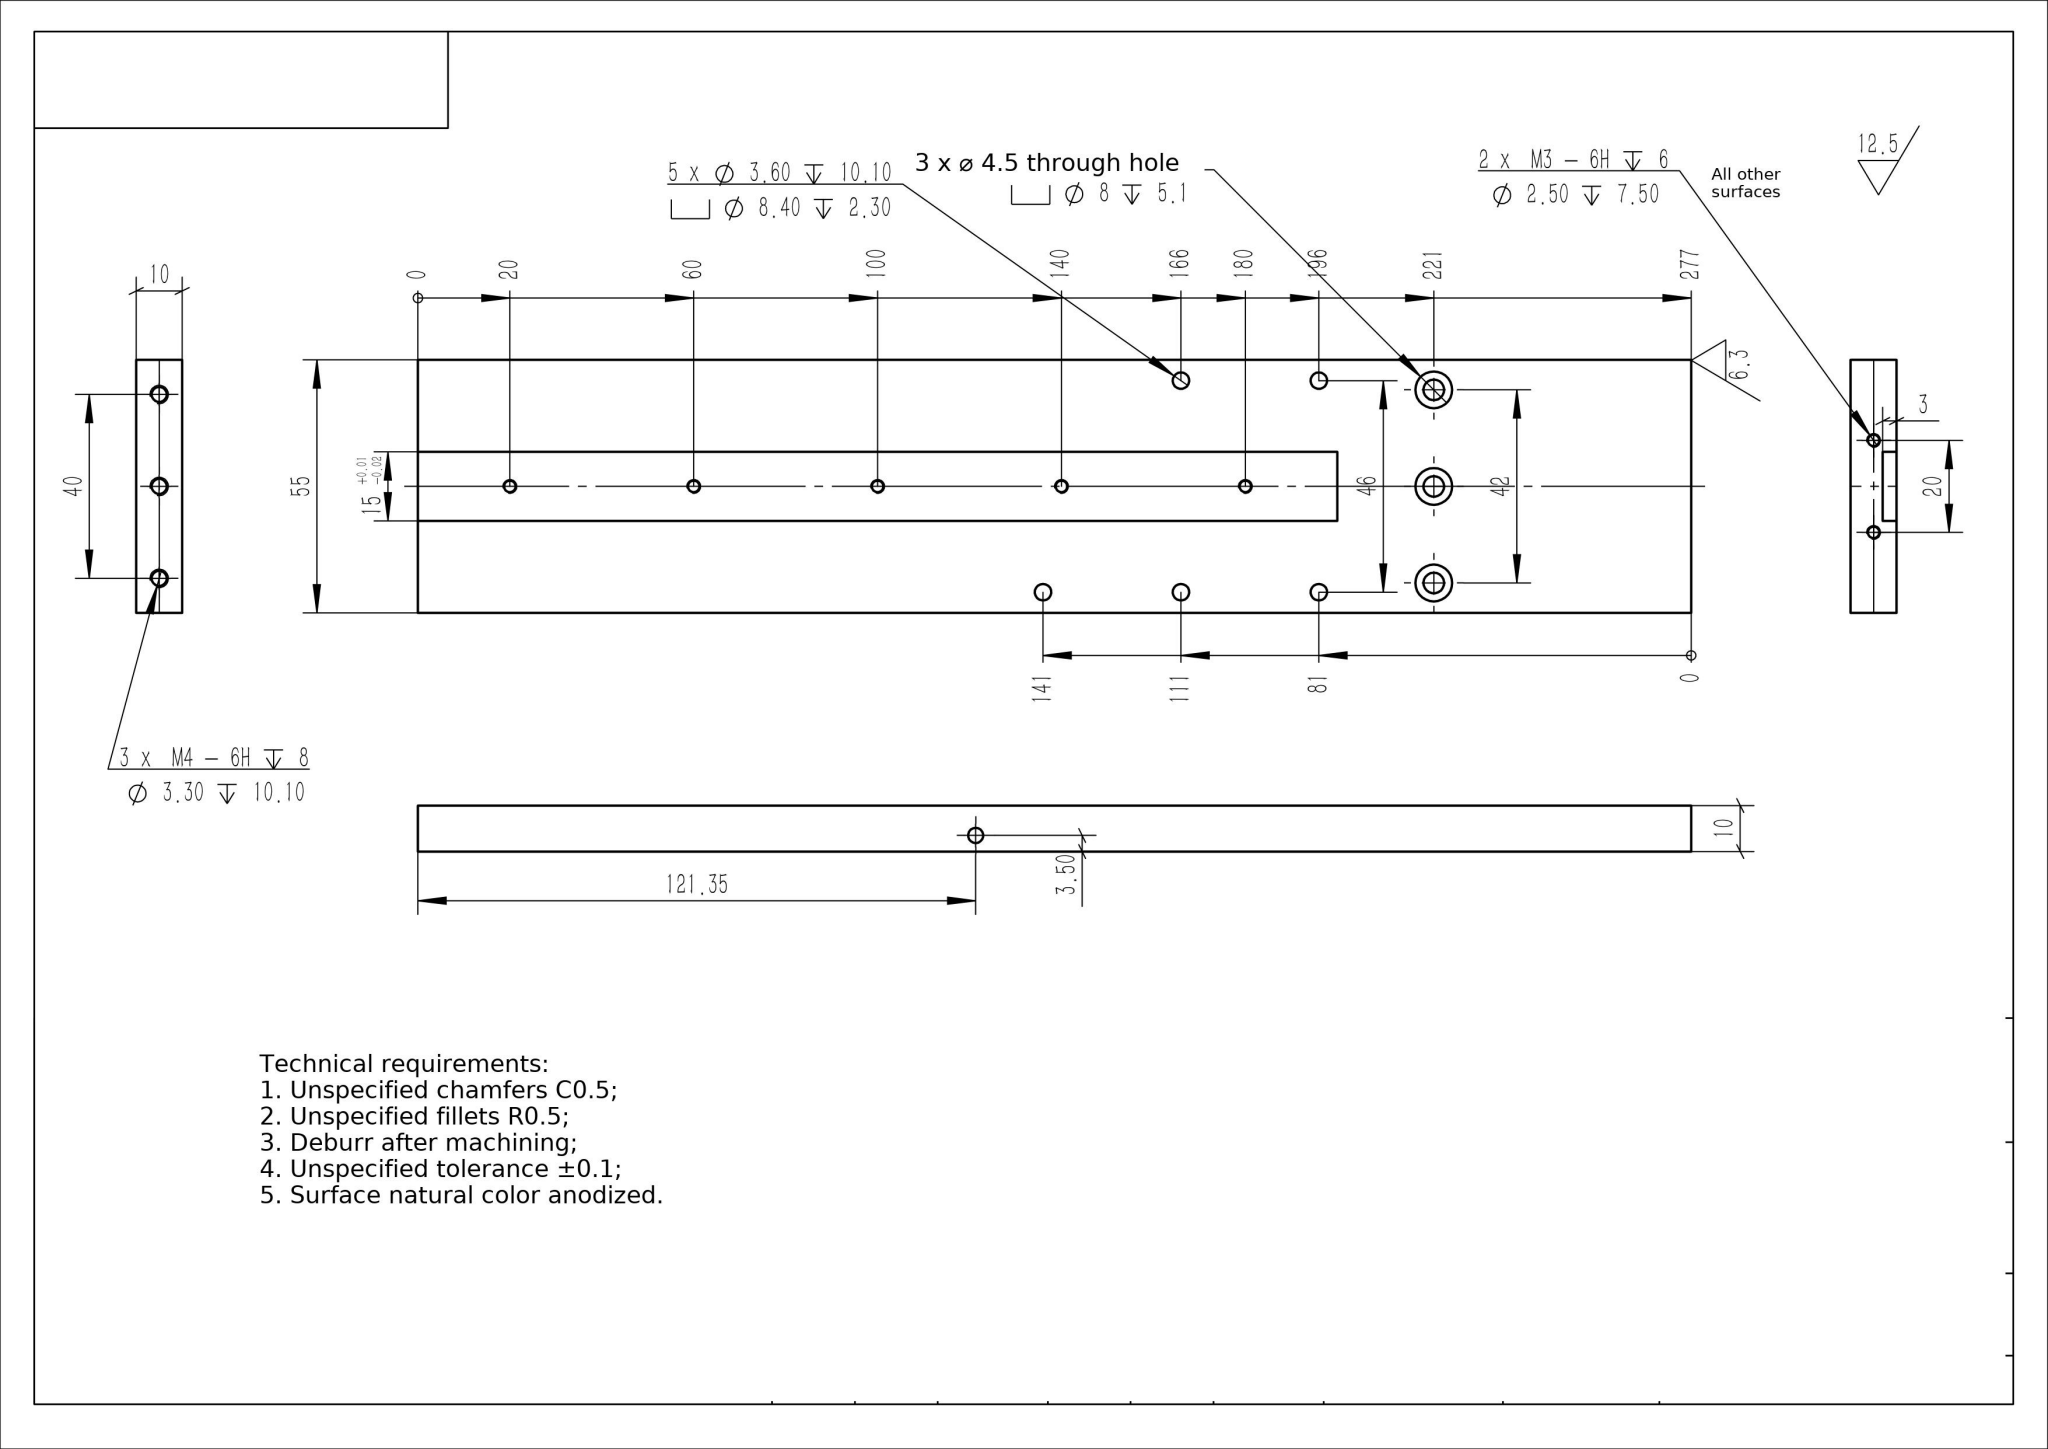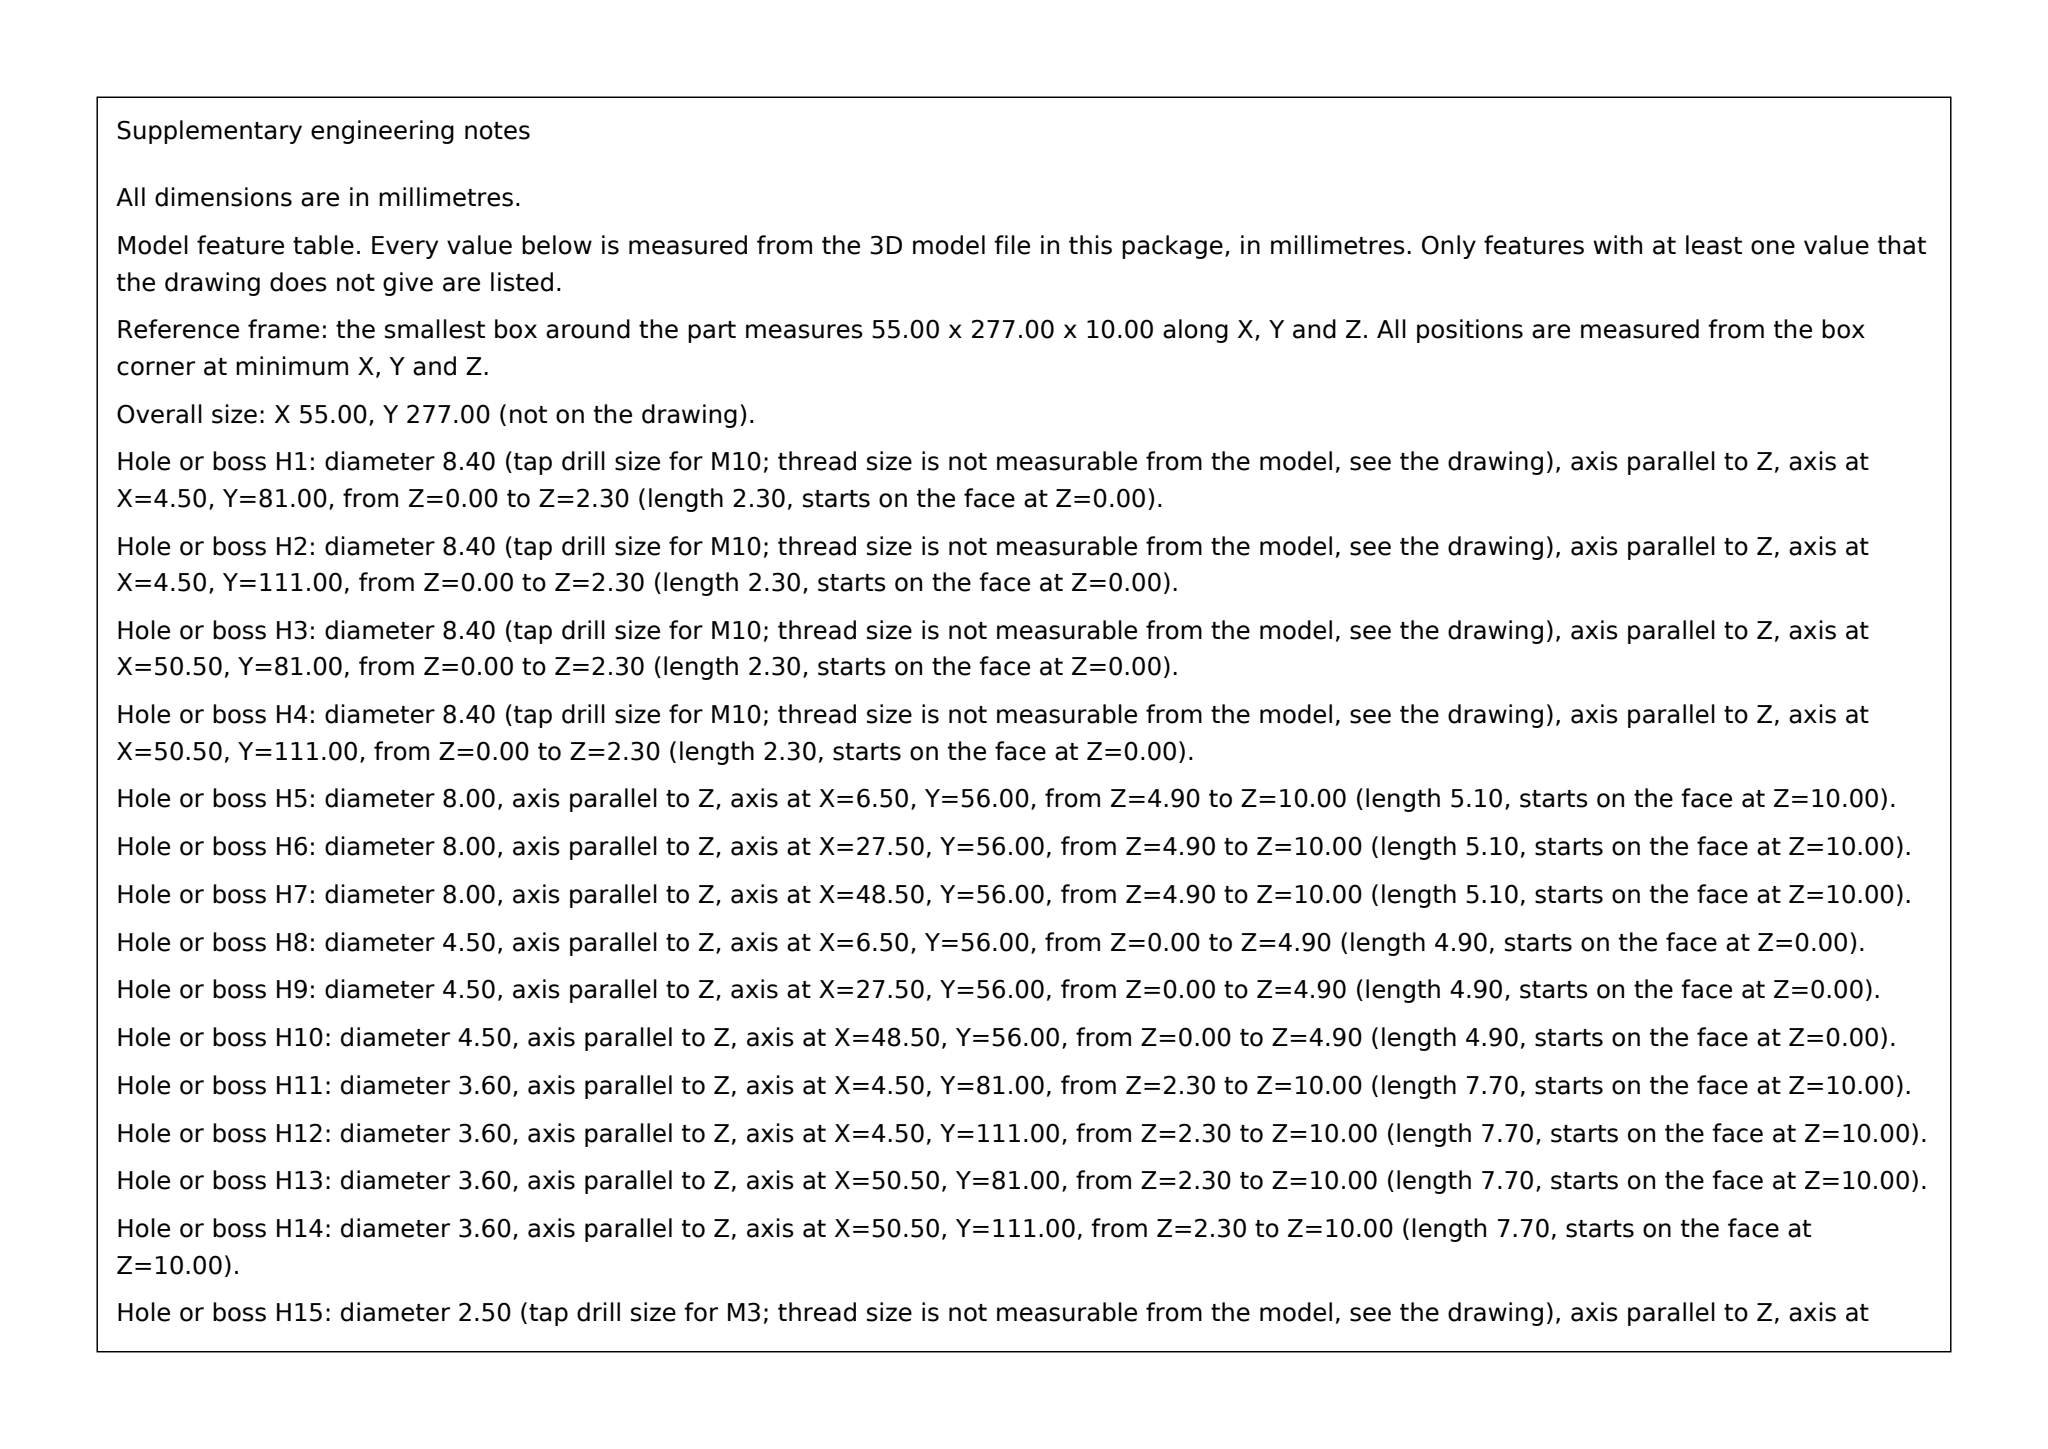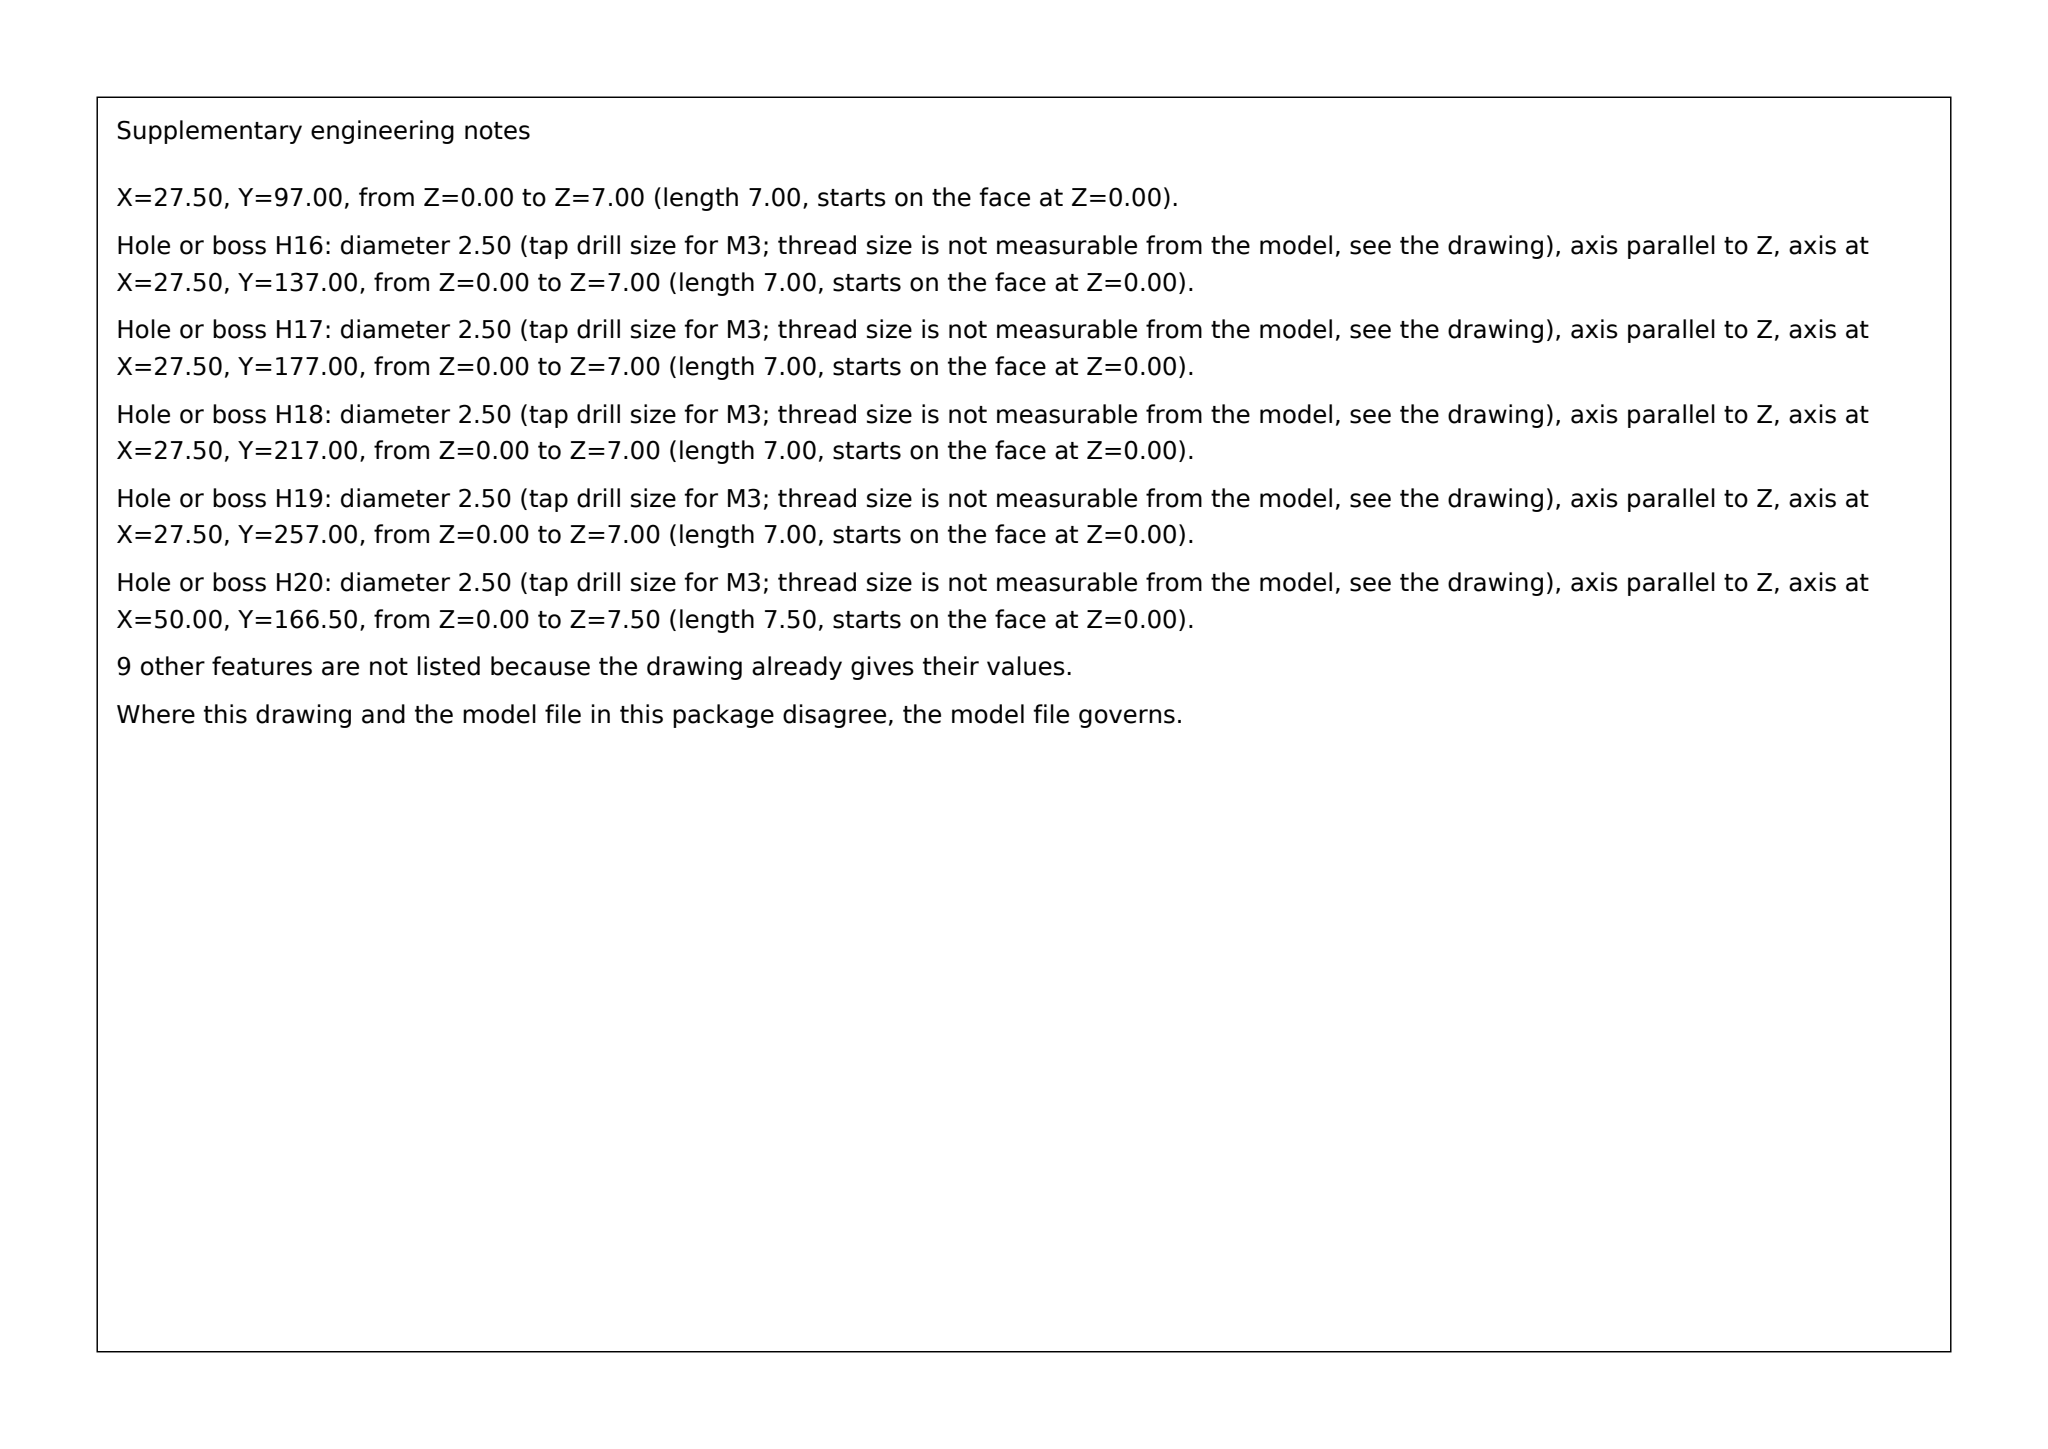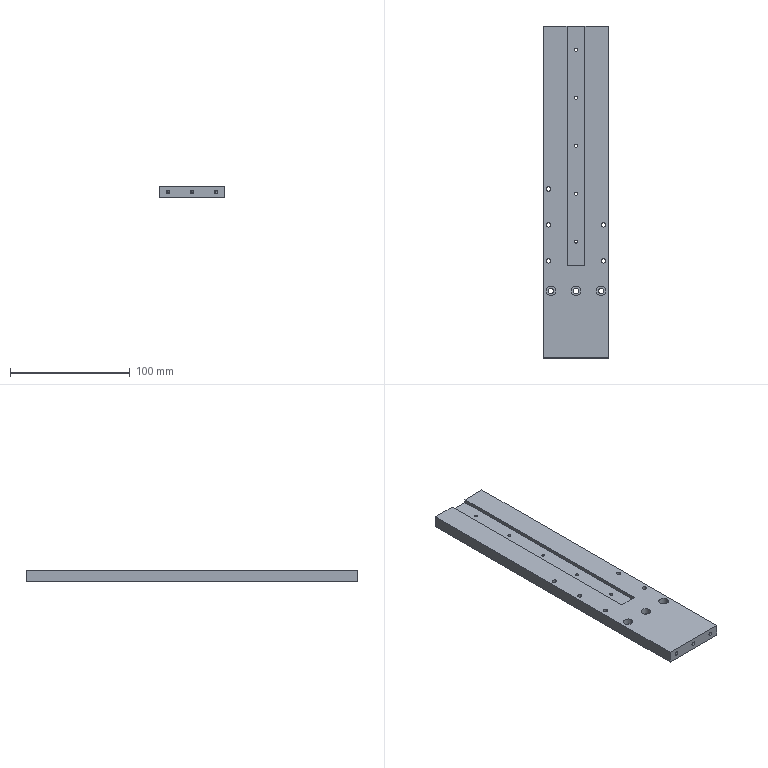Part | SolidWorks | mm | 1 solid | 92 faces | box 55 x 277 x 10 mm | volume 140637 mm3 | cylinder 58 | plane 18 | cone 16 | commonest cylinder face diameters 2.5 x18 8.4 x10 3.6 x10 3.3 x8 8 x6 4.5 x6
build123d program:
from build123d import *

# Parameters (mm, degrees)
SKETCH1_W                                           = 55
SKETCH1_H                                           = 277
BOSS_EXTRUDE1_DEPTH                                 = 10
HOLE_SIZE_ACCORDING_TO_HEXAGON_SOCKET_D             = 4.5
HOLE_SIZE_ACCORDING_TO_HEXAGON_SOCKET_CBORE_D       = 8
HOLE_SIZE_ACCORDING_TO_HEXAGON_SOCKET_CBORE_DEPTH   = 5.1
M4_TAPPED_HOLE1_D                                   = 3.3
M4_TAPPED_HOLE1_DEPTH                               = 10.1
M4_TAPPED_HOLE1_TIP                                 = 0.9914
M3_TAPPED_HOLE1_D                                   = 2.5
SKETCH21_W                                          = 15
SKETCH21_H                                          = 200
CUT_EXTRUDE2_DEPTH                                  = 3
M3_TAPPED_HOLE2_D                                   = 2.5
M3_TAPPED_HOLE2_DEPTH                               = 7.5
M3_TAPPED_HOLE2_TIP                                 = 0.7511
M4_TAPPED_HOLE2_D                                   = 3.3
M4_TAPPED_HOLE2_DEPTH                               = 10.1
M4_TAPPED_HOLE2_TIP                                 = 0.9914
M3_TAPPED_HOLE3_D                                   = 2.5
M3_TAPPED_HOLE3_DEPTH                               = 7.5
M3_TAPPED_HOLE3_TIP                                 = 0.7511
M3_HEX_HEAD_MACHINE_SCREW_COUNTERBORE_1_D           = 3.6
M3_HEX_HEAD_MACHINE_SCREW_COUNTERBORE_1_DEPTH       = 10.1
M3_HEX_HEAD_MACHINE_SCREW_COUNTERBORE_1_CBORE_D     = 8.4
M3_HEX_HEAD_MACHINE_SCREW_COUNTERBORE_1_CBORE_DEPTH = 2.3
M3_HEX_HEAD_MACHINE_SCREW_COUNTERBORE_1_TIP         = 1.082


with BuildPart() as part:
    # Sketch1 → Boss-Extrude1 (new body)
    with BuildSketch(Plane.XY):
        Rectangle(SKETCH1_W, SKETCH1_H)
    extrude(amount=BOSS_EXTRUDE1_DEPTH)

    # Hole Size _ according to_ Hexagon Socket (through all)
    with Locations(Plane.XY.offset(10)):
        with Locations((-21, -82.5), (0, -82.5), (21, -82.5)):
            CounterBoreHole(HOLE_SIZE_ACCORDING_TO_HEXAGON_SOCKET_D / 2, HOLE_SIZE_ACCORDING_TO_HEXAGON_SOCKET_CBORE_D / 2, HOLE_SIZE_ACCORDING_TO_HEXAGON_SOCKET_CBORE_DEPTH)

    # M4 Tapped Hole1
    with Locations(Plane(origin=(0, -138.5, 0), x_dir=(-1, 0, 0), z_dir=(0, -1, 0))):
        with Locations((20, -5), (-20, -5), (0, -5)):
            Hole(M4_TAPPED_HOLE1_D / 2, depth=M4_TAPPED_HOLE1_DEPTH)
            with Locations((0, 0, -(M4_TAPPED_HOLE1_DEPTH + M4_TAPPED_HOLE1_TIP / 2))):  # 118° drill point
                Cone(0, M4_TAPPED_HOLE1_D / 2, M4_TAPPED_HOLE1_TIP, mode=Mode.SUBTRACT)

    # M3 Tapped Hole1 (through all)
    with Locations(Plane.XY.offset(10)):
        with Locations((0, 118.5), (0, 78.5), (0, 38.5), (0, -1.5), (0, -41.5)):
            Hole(M3_TAPPED_HOLE1_D / 2)

    # Sketch21 → Cut-Extrude2 (cut)
    with BuildSketch(Plane.XY.offset(10)):
        with Locations((0, 38.5)):
            Rectangle(SKETCH21_W, SKETCH21_H)
    extrude(amount=-CUT_EXTRUDE2_DEPTH, mode=Mode.SUBTRACT)

    # M3 Tapped Hole2
    with Locations(Plane(origin=(0, 138.5, 0), x_dir=(1, 0, 0), z_dir=(0, 1, 0))):
        with Locations((-10, -5), (10, -5)):
            Hole(M3_TAPPED_HOLE2_D / 2, depth=M3_TAPPED_HOLE2_DEPTH)
            with Locations((0, 0, -(M3_TAPPED_HOLE2_DEPTH + M3_TAPPED_HOLE2_TIP / 2))):  # 118° drill point
                Cone(0, M3_TAPPED_HOLE2_D / 2, M3_TAPPED_HOLE2_TIP, mode=Mode.SUBTRACT)

    # M4 Tapped Hole2
    with Locations(Plane(origin=(27.5, 0, 0), x_dir=(0, 0, -1), z_dir=(1, 0, 0))):
        with Locations((-6.5, 17.15)):
            Hole(M4_TAPPED_HOLE2_D / 2, depth=M4_TAPPED_HOLE2_DEPTH)
            with Locations((0, 0, -(M4_TAPPED_HOLE2_DEPTH + M4_TAPPED_HOLE2_TIP / 2))):  # 118° drill point
                Cone(0, M4_TAPPED_HOLE2_D / 2, M4_TAPPED_HOLE2_TIP, mode=Mode.SUBTRACT)

    # M3 Tapped Hole3
    with Locations(Plane(origin=(0, 0, 0), x_dir=(-1, 0, 0), z_dir=(0, 0, -1))):
        with Locations((-22.5, 28), (-22.5, 3)):
            Hole(M3_TAPPED_HOLE3_D / 2, depth=M3_TAPPED_HOLE3_DEPTH)
            with Locations((0, 0, -(M3_TAPPED_HOLE3_DEPTH + M3_TAPPED_HOLE3_TIP / 2))):  # 118° drill point
                Cone(0, M3_TAPPED_HOLE3_D / 2, M3_TAPPED_HOLE3_TIP, mode=Mode.SUBTRACT)

    # M3 Hex Head Machine Screw Counterbore 1
    with Locations(Plane(origin=(0, 0, 0), x_dir=(-1, 0, 0), z_dir=(0, 0, -1))):
        with Locations((-23, -27.5), (-23, -57.5), (23, 2.5), (23, -27.5), (23, -57.5)):
            CounterBoreHole(M3_HEX_HEAD_MACHINE_SCREW_COUNTERBORE_1_D / 2, M3_HEX_HEAD_MACHINE_SCREW_COUNTERBORE_1_CBORE_D / 2, M3_HEX_HEAD_MACHINE_SCREW_COUNTERBORE_1_CBORE_DEPTH, depth=M3_HEX_HEAD_MACHINE_SCREW_COUNTERBORE_1_DEPTH)
            with Locations((0, 0, -(M3_HEX_HEAD_MACHINE_SCREW_COUNTERBORE_1_DEPTH + M3_HEX_HEAD_MACHINE_SCREW_COUNTERBORE_1_TIP / 2))):  # 118° drill point
                Cone(0, M3_HEX_HEAD_MACHINE_SCREW_COUNTERBORE_1_D / 2, M3_HEX_HEAD_MACHINE_SCREW_COUNTERBORE_1_TIP, mode=Mode.SUBTRACT)


solid = part.part